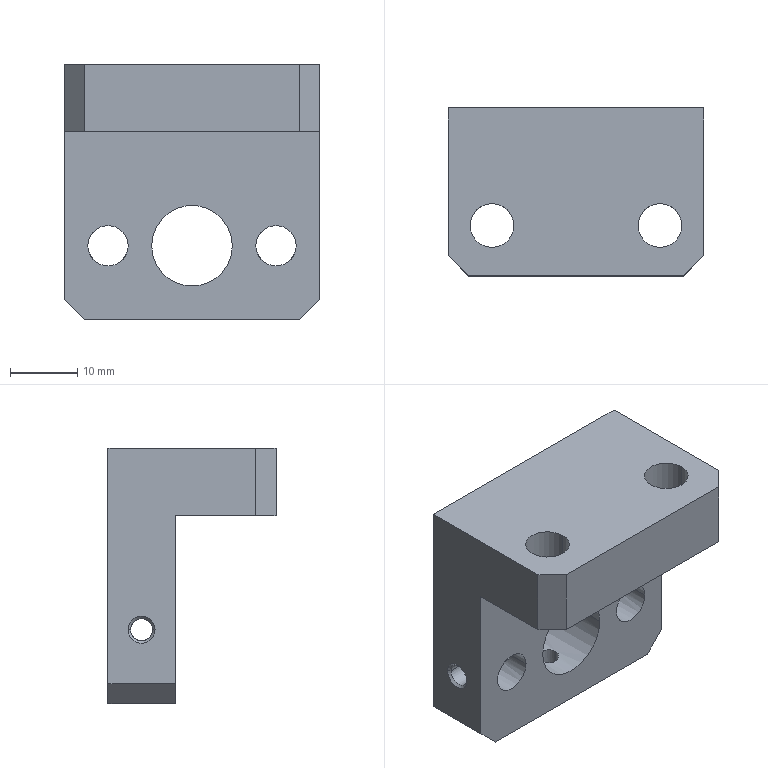Component | SolidWorks | GluePaperFeedingTensioningWheelAssembly-1_YX-04-113GluePaperFeedingTensioningWheelFixingBlock-1 | 1 solid | 38 faces | volume 17430 mm3 | cylinder 20 | plane 12 | cone 6 | commonest cylinder face diameters 3.3 x10 6.5 x4 6 x4 12 x2 | material 45#Steel